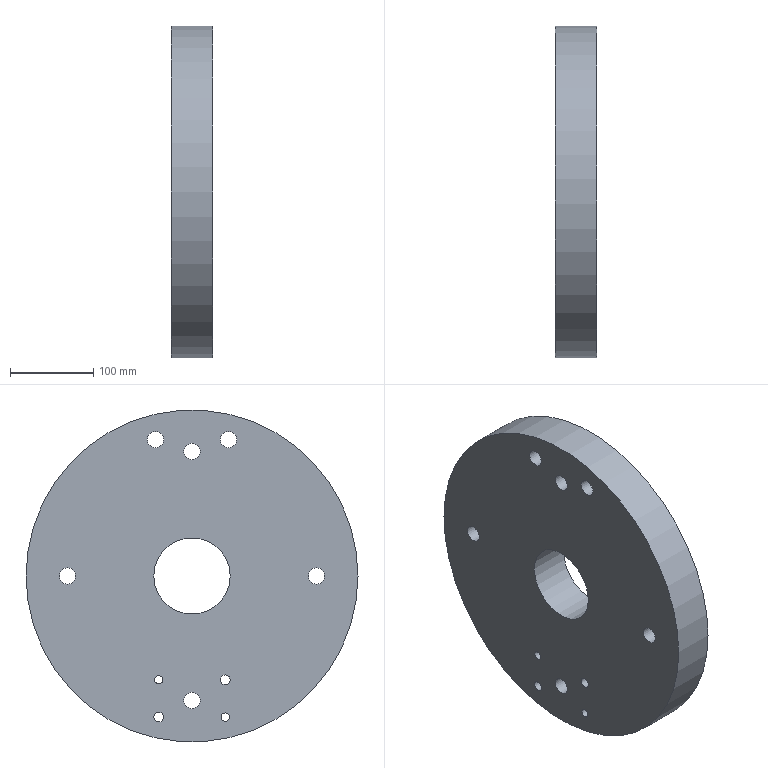Component | NX | FACEPLATE | 1 solid | 14 faces | volume 5841470 mm3 | cylinder 12 | plane 2 | commonest cylinder face diameters 19.623 x6 10 x2 11.701 x2 400 x1 92 x1